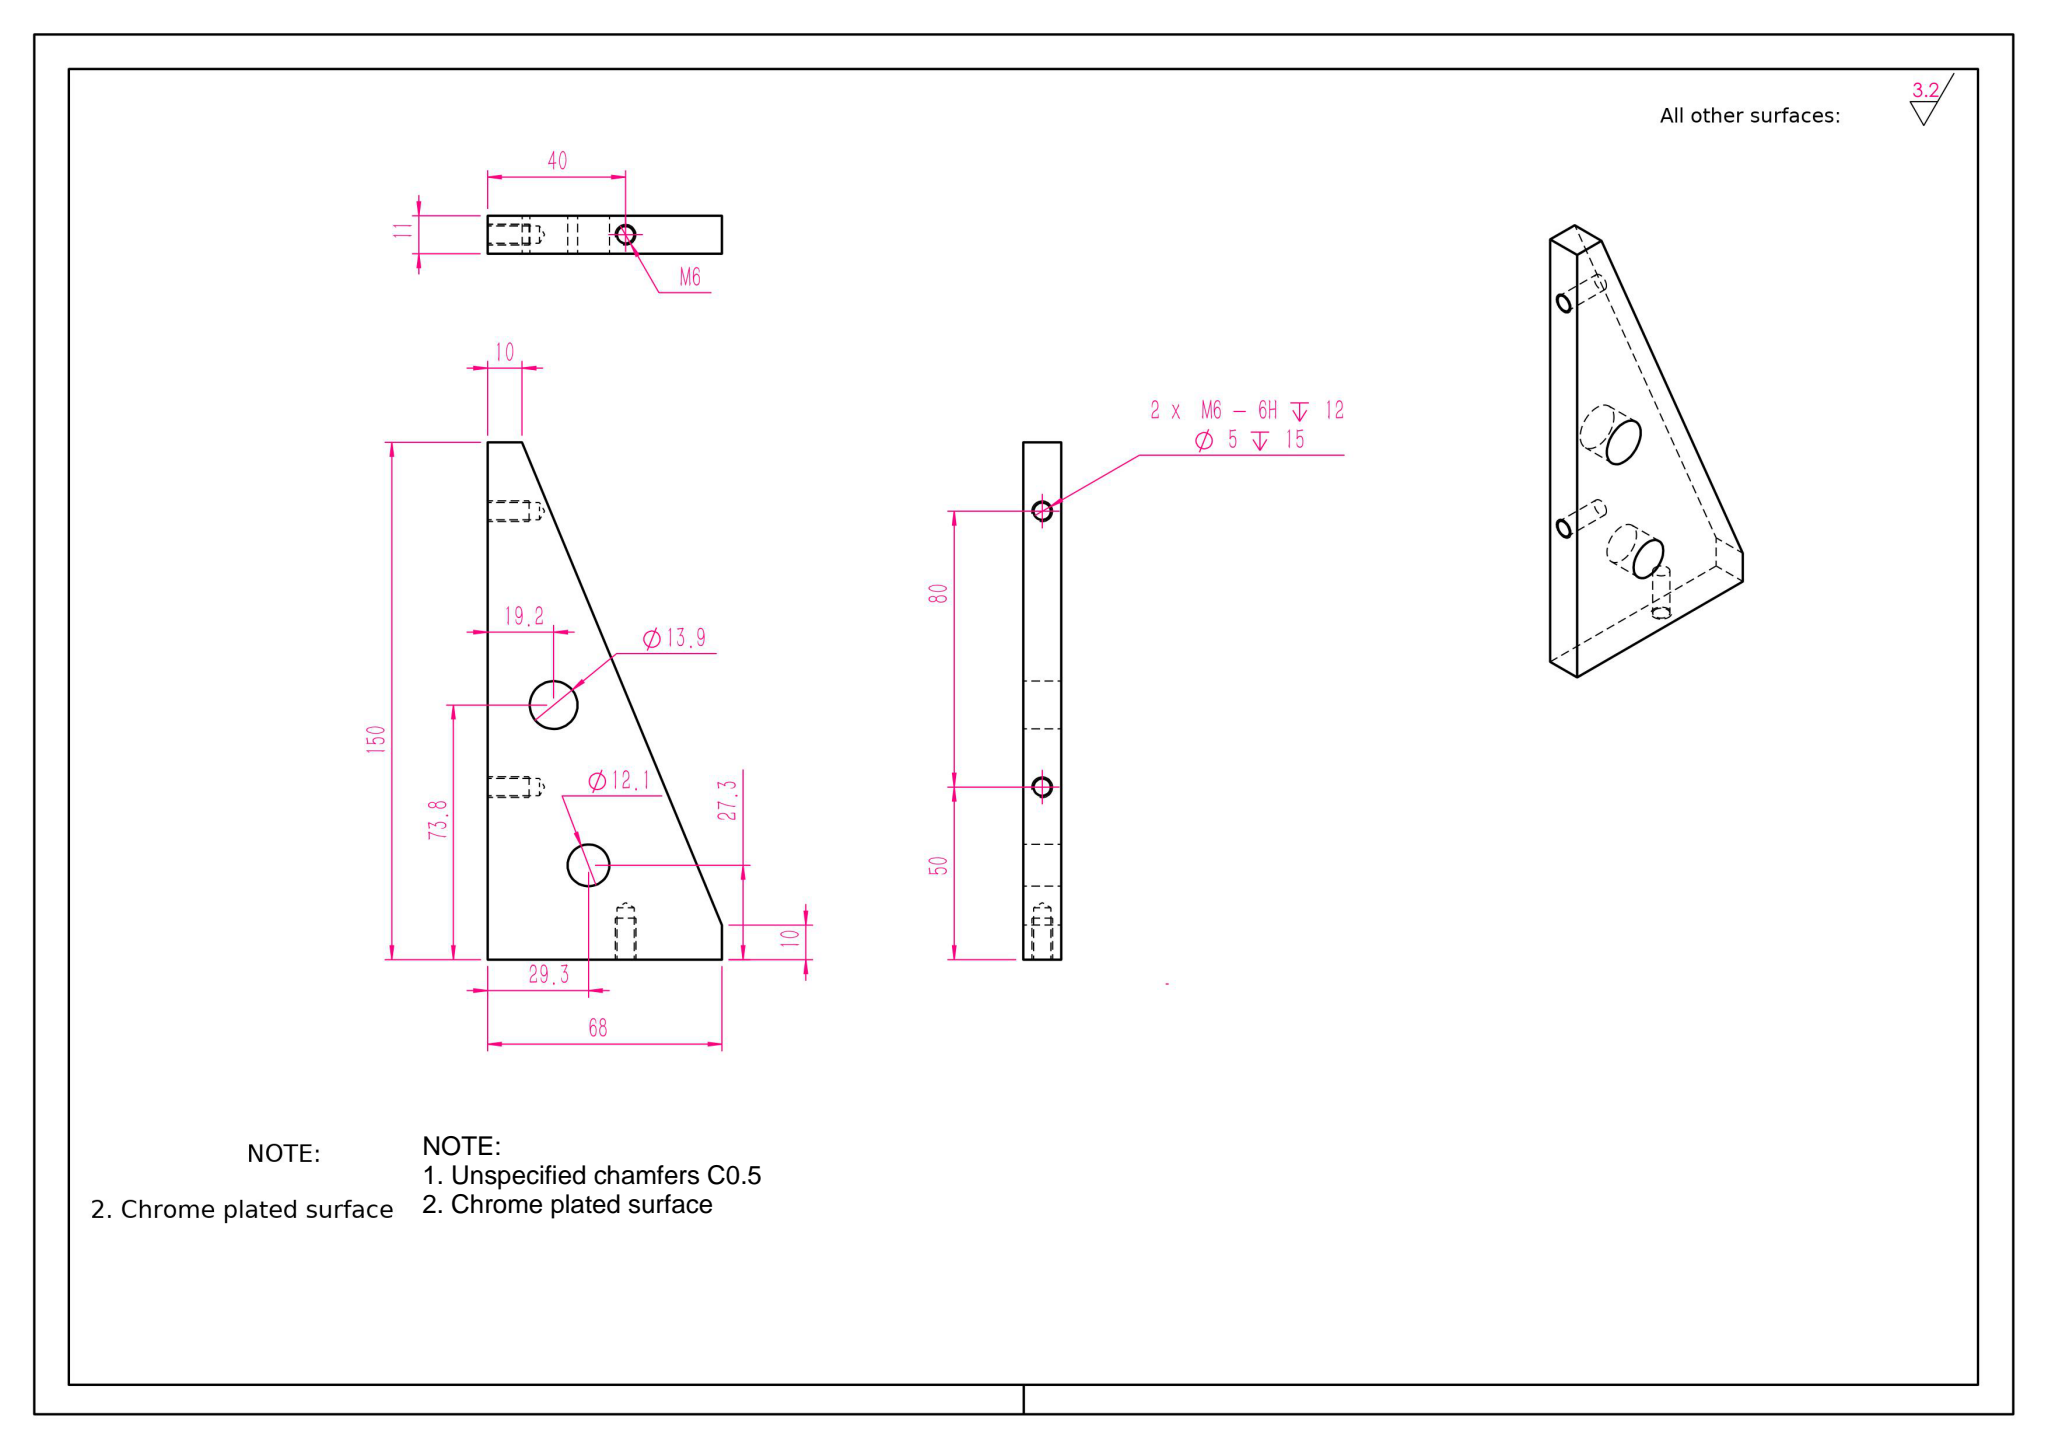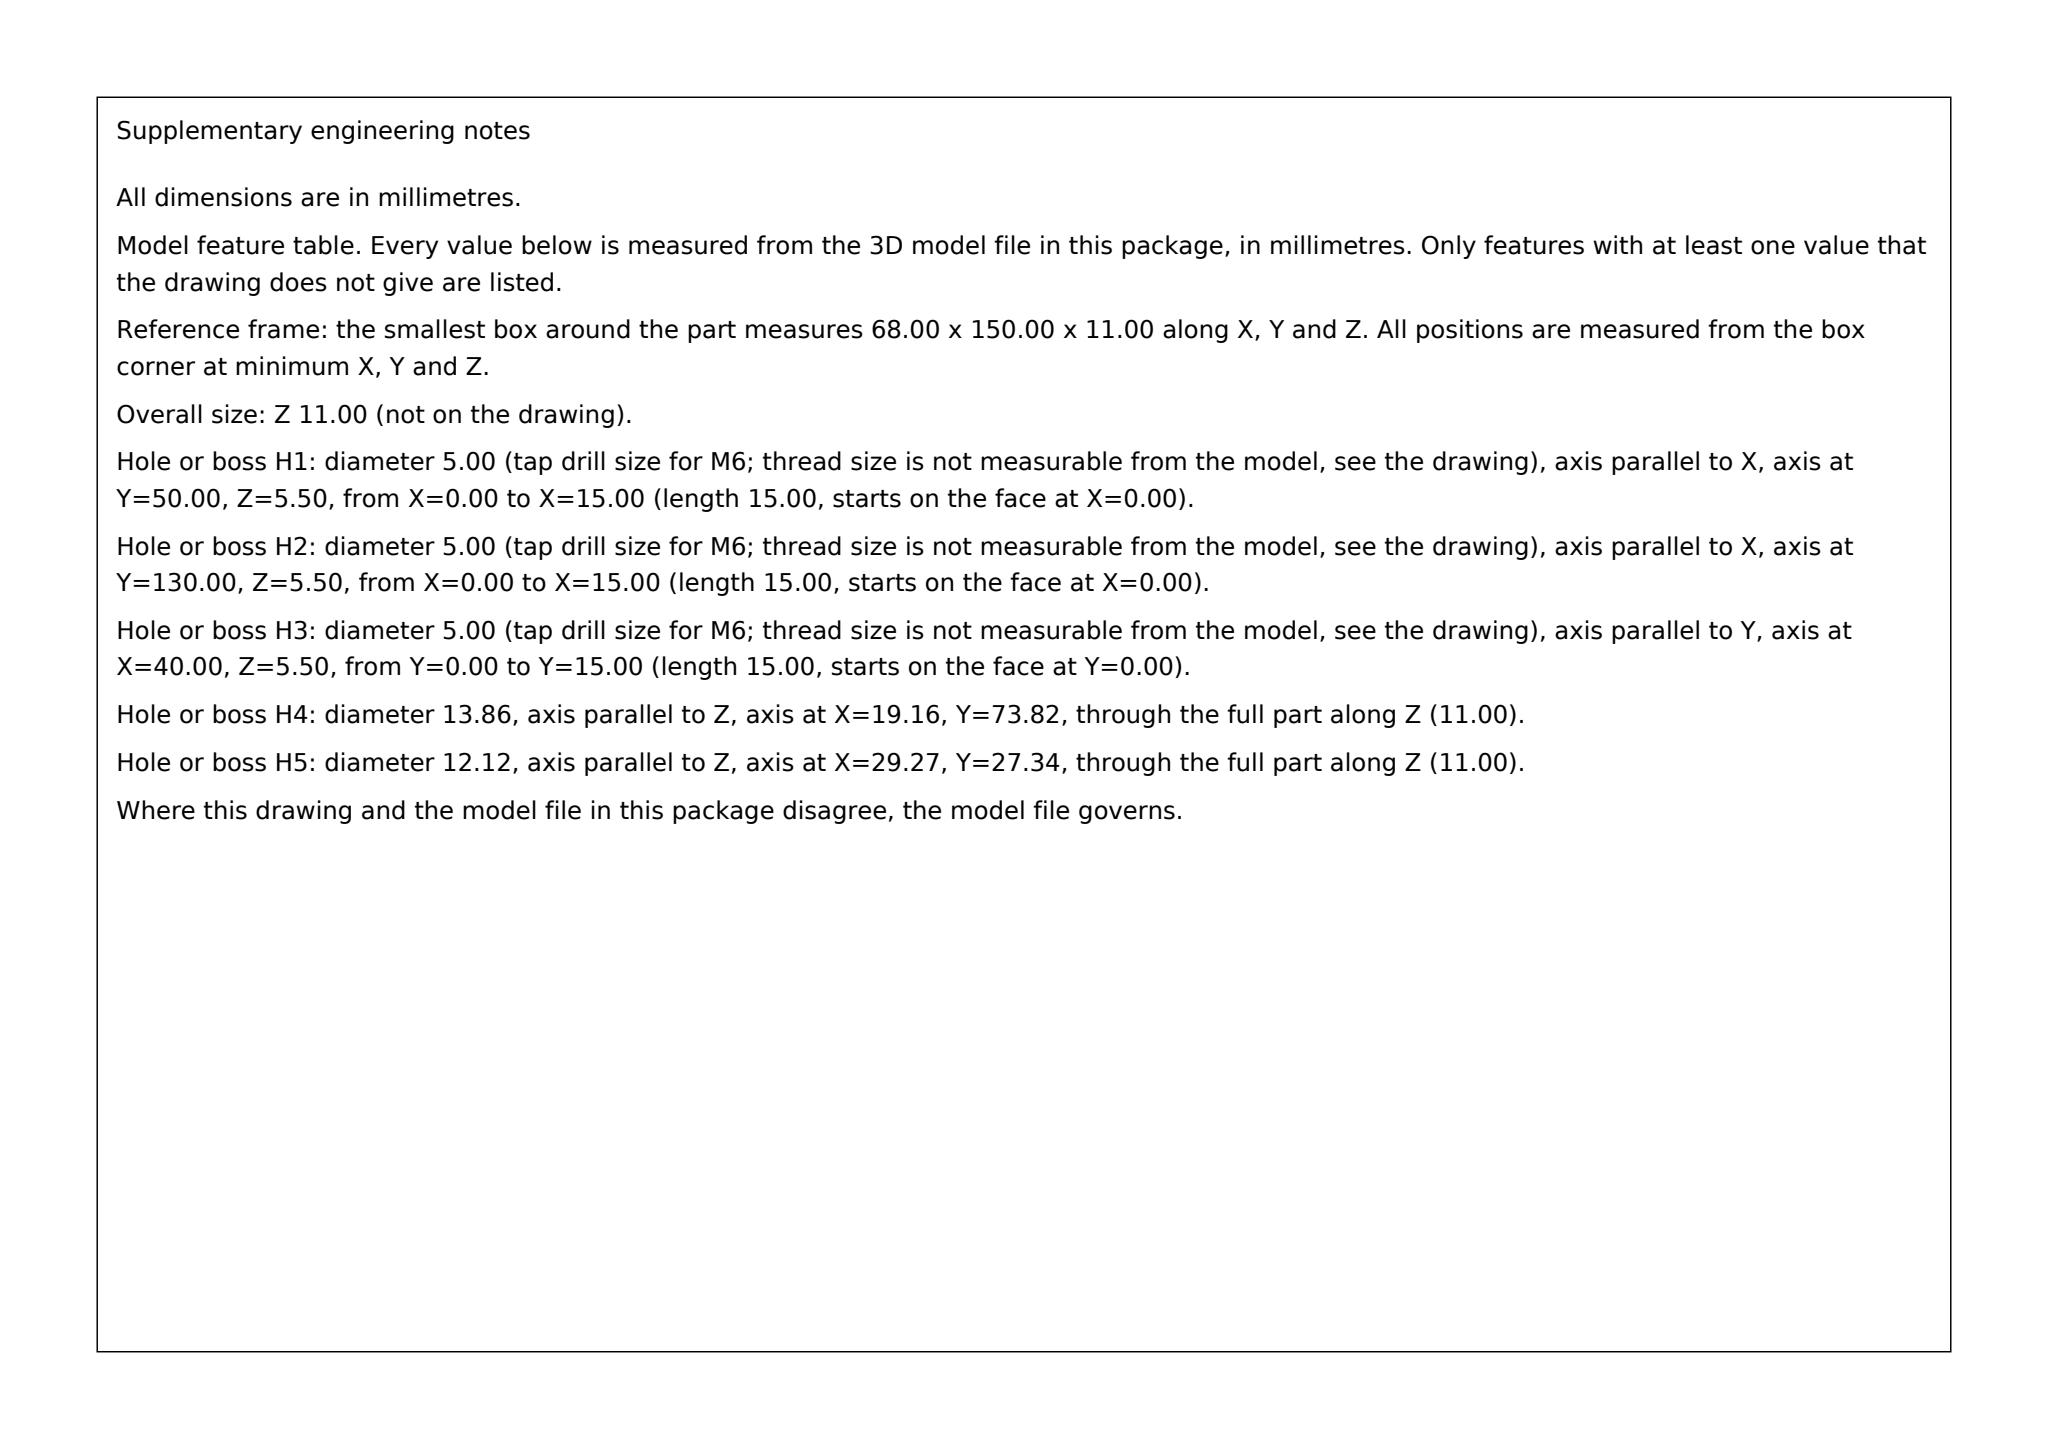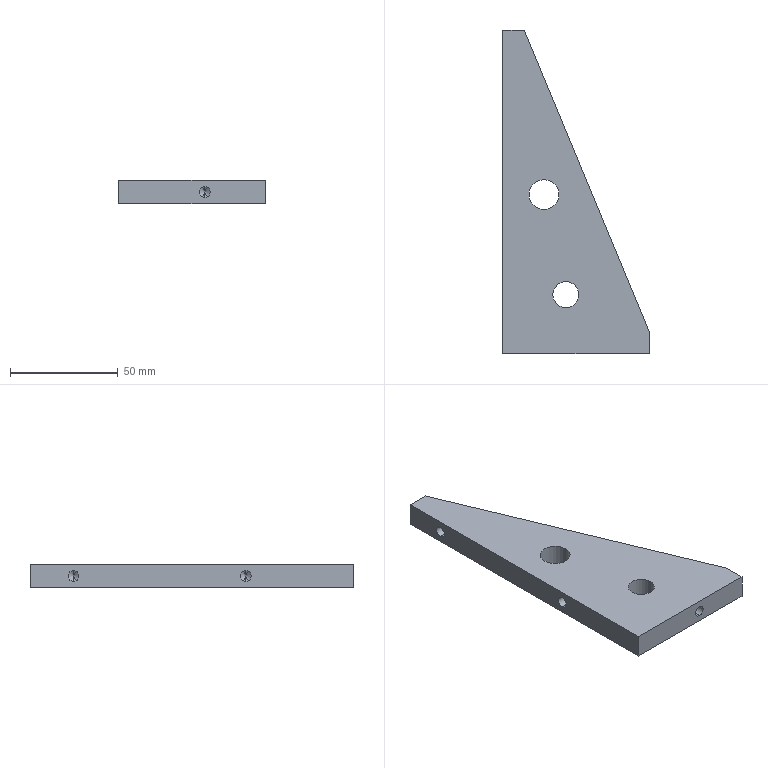Part | SolidWorks | mm | 1 solid | 23 faces | box 68 x 150 x 11 mm | volume 63698 mm3 | cylinder 10 | plane 7 | cone 6 | commonest cylinder face diameters 5 x6 12.125 x2 13.857 x2
build123d program:
from build123d import *

# Parameters (mm, degrees)
BOSS_EXTRUDE1_DEPTH   = 11
M6_TAPPED_HOLE1_D     = 5
M6_TAPPED_HOLE1_DEPTH = 15
M6_TAPPED_HOLE1_TIP   = 1.502
M6_TAPPED_HOLE2_D     = 5
M6_TAPPED_HOLE2_DEPTH = 15
M6_TAPPED_HOLE2_TIP   = 1.502
SKETCH8_R             = 6.063
SKETCH8_R_2           = 6.928
CUT_EXTRUDE1_DEPTH    = 80


with BuildPart() as part:
    # Sketch1 → Boss-Extrude1 (new body)
    with BuildSketch(Plane.XY):
        Polygon((0, 0), (68, 0), (68, 10), (10, 150), (0, 150), align=None)
    extrude(amount=BOSS_EXTRUDE1_DEPTH)

    # M6 Tapped Hole1
    with Locations(Plane(origin=(0, 0, 0), x_dir=(-1, 0, 0), z_dir=(0, -1, 0))):
        with Locations((-40, -5.5)):
            Hole(M6_TAPPED_HOLE1_D / 2, depth=M6_TAPPED_HOLE1_DEPTH)
            with Locations((0, 0, -(M6_TAPPED_HOLE1_DEPTH + M6_TAPPED_HOLE1_TIP / 2))):  # 118° drill point
                Cone(0, M6_TAPPED_HOLE1_D / 2, M6_TAPPED_HOLE1_TIP, mode=Mode.SUBTRACT)

    # M6 Tapped Hole2
    with Locations(Plane.ZY):
        with Locations((5.5, 130), (5.5, 50)):
            Hole(M6_TAPPED_HOLE2_D / 2, depth=M6_TAPPED_HOLE2_DEPTH)
            with Locations((0, 0, -(M6_TAPPED_HOLE2_DEPTH + M6_TAPPED_HOLE2_TIP / 2))):  # 118° drill point
                Cone(0, M6_TAPPED_HOLE2_D / 2, M6_TAPPED_HOLE2_TIP, mode=Mode.SUBTRACT)

    # Sketch8 → Cut-Extrude1 (cut)
    with BuildSketch(Plane.XY.offset(11)):
        with Locations((29.268, 27.343)):
            Circle(SKETCH8_R)
        with Locations((19.156, 73.817)):
            Circle(SKETCH8_R_2)
    extrude(amount=-CUT_EXTRUDE1_DEPTH, mode=Mode.SUBTRACT)


solid = part.part
STEP:
#1=CARTESIAN_POINT('',(23.206,27.343,0.));
#2=VERTEX_POINT('',#1);
#3=CARTESIAN_POINT('',(35.331,27.343,0.));
#4=VERTEX_POINT('',#3);
#5=CARTESIAN_POINT('',(29.268,27.343,0.));
#6=DIRECTION('',(0.,0.,1.));
#7=DIRECTION('',(1.,0.,0.));
#8=AXIS2_PLACEMENT_3D('',#5,#6,#7);
#9=CIRCLE('',#8,6.063);
#10=EDGE_CURVE('',#2,#4,#9,.T.);
#11=ORIENTED_EDGE('',*,*,#10,.F.);
#12=CARTESIAN_POINT('',(23.206,27.343,11.));
#13=VERTEX_POINT('',#12);
#14=CARTESIAN_POINT('',(23.206,27.343,-69.));
#15=DIRECTION('',(0.,0.,1.));
#16=VECTOR('',#15,1000.);
#17=LINE('',#14,#16);
#18=EDGE_CURVE('',#2,#13,#17,.T.);
#19=ORIENTED_EDGE('',*,*,#18,.T.);
#20=CARTESIAN_POINT('',(35.331,27.343,11.));
#21=VERTEX_POINT('',#20);
#22=CARTESIAN_POINT('',(29.268,27.343,11.));
#23=DIRECTION('',(0.,0.,1.));
#24=DIRECTION('',(1.,0.,0.));
#25=AXIS2_PLACEMENT_3D('',#22,#23,#24);
#26=CIRCLE('',#25,6.063);
#27=EDGE_CURVE('',#13,#21,#26,.T.);
#28=ORIENTED_EDGE('',*,*,#27,.T.);
#29=CARTESIAN_POINT('',(35.331,27.343,-69.));
#30=DIRECTION('',(0.,0.,1.));
#31=VECTOR('',#30,1000.);
#32=LINE('',#29,#31);
#33=EDGE_CURVE('',#4,#21,#32,.T.);
#34=ORIENTED_EDGE('',*,*,#33,.F.);
#35=EDGE_LOOP('',(#11,#19,#28,#34));
#36=FACE_OUTER_BOUND('',#35,.T.);
#37=CARTESIAN_POINT('',(29.268,27.343,-69.));
#38=DIRECTION('',(0.,0.,1.));
#39=DIRECTION('',(1.,0.,0.));
#40=AXIS2_PLACEMENT_3D('',#37,#38,#39);
#41=CYLINDRICAL_SURFACE('',#40,6.063);
#42=ADVANCED_FACE('',(#36),#41,.F.);
#43=CARTESIAN_POINT('',(12.228,73.817,0.));
#44=VERTEX_POINT('',#43);
#45=CARTESIAN_POINT('',(26.085,73.817,0.));
#46=VERTEX_POINT('',#45);
#47=CARTESIAN_POINT('',(19.156,73.817,0.));
#48=DIRECTION('',(0.,0.,1.));
#49=DIRECTION('',(1.,0.,0.));
#50=AXIS2_PLACEMENT_3D('',#47,#48,#49);
#51=CIRCLE('',#50,6.928);
#52=EDGE_CURVE('',#44,#46,#51,.T.);
#53=ORIENTED_EDGE('',*,*,#52,.F.);
#54=CARTESIAN_POINT('',(12.228,73.817,11.));
#55=VERTEX_POINT('',#54);
#56=CARTESIAN_POINT('',(12.228,73.817,-69.));
#57=DIRECTION('',(0.,0.,1.));
#58=VECTOR('',#57,1000.);
#59=LINE('',#56,#58);
#60=EDGE_CURVE('',#44,#55,#59,.T.);
#61=ORIENTED_EDGE('',*,*,#60,.T.);
#62=CARTESIAN_POINT('',(26.085,73.817,11.));
#63=VERTEX_POINT('',#62);
#64=CARTESIAN_POINT('',(19.156,73.817,11.));
#65=DIRECTION('',(0.,0.,1.));
#66=DIRECTION('',(1.,0.,0.));
#67=AXIS2_PLACEMENT_3D('',#64,#65,#66);
#68=CIRCLE('',#67,6.928);
#69=EDGE_CURVE('',#55,#63,#68,.T.);
#70=ORIENTED_EDGE('',*,*,#69,.T.);
#71=CARTESIAN_POINT('',(26.085,73.817,-69.));
#72=DIRECTION('',(0.,0.,1.));
#73=VECTOR('',#72,1000.);
#74=LINE('',#71,#73);
#75=EDGE_CURVE('',#46,#63,#74,.T.);
#76=ORIENTED_EDGE('',*,*,#75,.F.);
#77=EDGE_LOOP('',(#53,#61,#70,#76));
#78=FACE_OUTER_BOUND('',#77,.T.);
#79=CARTESIAN_POINT('',(19.156,73.817,-69.));
#80=DIRECTION('',(0.,0.,1.));
#81=DIRECTION('',(1.,0.,0.));
#82=AXIS2_PLACEMENT_3D('',#79,#80,#81);
#83=CYLINDRICAL_SURFACE('',#82,6.928);
#84=ADVANCED_FACE('',(#78),#83,.F.);
#85=CARTESIAN_POINT('',(15.,130.,3.));
#86=VERTEX_POINT('',#85);
#87=CARTESIAN_POINT('',(15.,130.,8.));
#88=VERTEX_POINT('',#87);
#89=CARTESIAN_POINT('',(15.,130.,5.5));
#90=DIRECTION('',(-1.,0.,0.));
#91=DIRECTION('',(0.,0.,1.));
#92=AXIS2_PLACEMENT_3D('',#89,#90,#91);
#93=CIRCLE('',#92,2.5);
#94=EDGE_CURVE('',#86,#88,#93,.T.);
#95=ORIENTED_EDGE('',*,*,#94,.F.);
#96=CARTESIAN_POINT('',(-0.,130.,3.));
#97=VERTEX_POINT('',#96);
#98=CARTESIAN_POINT('',(-0.,130.,3.));
#99=DIRECTION('',(-1.,0.,0.));
#100=VECTOR('',#99,1000.);
#101=LINE('',#98,#100);
#102=EDGE_CURVE('',#86,#97,#101,.T.);
#103=ORIENTED_EDGE('',*,*,#102,.T.);
#104=CARTESIAN_POINT('',(-0.,130.,8.));
#105=VERTEX_POINT('',#104);
#106=CARTESIAN_POINT('',(-0.,130.,5.5));
#107=DIRECTION('',(-1.,0.,0.));
#108=DIRECTION('',(0.,0.,1.));
#109=AXIS2_PLACEMENT_3D('',#106,#107,#108);
#110=CIRCLE('',#109,2.5);
#111=EDGE_CURVE('',#97,#105,#110,.T.);
#112=ORIENTED_EDGE('',*,*,#111,.T.);
#113=CARTESIAN_POINT('',(-0.,130.,8.));
#114=DIRECTION('',(-1.,0.,0.));
#115=VECTOR('',#114,1000.);
#116=LINE('',#113,#115);
#117=EDGE_CURVE('',#88,#105,#116,.T.);
#118=ORIENTED_EDGE('',*,*,#117,.F.);
#119=EDGE_LOOP('',(#95,#103,#112,#118));
#120=FACE_OUTER_BOUND('',#119,.T.);
#121=CARTESIAN_POINT('',(-0.,130.,5.5));
#122=DIRECTION('',(-1.,0.,0.));
#123=DIRECTION('',(0.,0.,1.));
#124=AXIS2_PLACEMENT_3D('',#121,#122,#123);
#125=CYLINDRICAL_SURFACE('',#124,2.5);
#126=ADVANCED_FACE('',(#120),#125,.F.);
#127=CARTESIAN_POINT('',(16.502,130.,5.5));
#128=VERTEX_POINT('',#127);
#129=CARTESIAN_POINT('',(15.,130.,8.));
#130=DIRECTION('',(-0.515,0.,0.8572));
#131=VECTOR('',#130,1000.);
#132=LINE('',#129,#131);
#133=EDGE_CURVE('',#128,#88,#132,.T.);
#134=ORIENTED_EDGE('',*,*,#133,.F.);
#135=CARTESIAN_POINT('',(15.,130.,3.));
#136=DIRECTION('',(-0.515,0.,-0.8572));
#137=VECTOR('',#136,1000.);
#138=LINE('',#135,#137);
#139=EDGE_CURVE('',#128,#86,#138,.T.);
#140=ORIENTED_EDGE('',*,*,#139,.T.);
#141=ORIENTED_EDGE('',*,*,#94,.T.);
#142=EDGE_LOOP('',(#134,#140,#141));
#143=FACE_OUTER_BOUND('',#142,.T.);
#144=CARTESIAN_POINT('',(15.,130.,5.5));
#145=DIRECTION('',(-1.,0.,0.));
#146=DIRECTION('',(0.,0.,1.));
#147=AXIS2_PLACEMENT_3D('',#144,#145,#146);
#148=CONICAL_SURFACE('',#147,2.5,1.03);
#149=ADVANCED_FACE('',(#143),#148,.F.);
#150=CARTESIAN_POINT('',(15.,50.,3.));
#151=VERTEX_POINT('',#150);
#152=CARTESIAN_POINT('',(15.,50.,8.));
#153=VERTEX_POINT('',#152);
#154=CARTESIAN_POINT('',(15.,50.,5.5));
#155=DIRECTION('',(-1.,0.,0.));
#156=DIRECTION('',(0.,0.,1.));
#157=AXIS2_PLACEMENT_3D('',#154,#155,#156);
#158=CIRCLE('',#157,2.5);
#159=EDGE_CURVE('',#151,#153,#158,.T.);
#160=ORIENTED_EDGE('',*,*,#159,.F.);
#161=CARTESIAN_POINT('',(-0.,50.,3.));
#162=VERTEX_POINT('',#161);
#163=CARTESIAN_POINT('',(-0.,50.,3.));
#164=DIRECTION('',(-1.,0.,0.));
#165=VECTOR('',#164,1000.);
#166=LINE('',#163,#165);
#167=EDGE_CURVE('',#151,#162,#166,.T.);
#168=ORIENTED_EDGE('',*,*,#167,.T.);
#169=CARTESIAN_POINT('',(-0.,50.,8.));
#170=VERTEX_POINT('',#169);
#171=CARTESIAN_POINT('',(-0.,50.,5.5));
#172=DIRECTION('',(-1.,0.,0.));
#173=DIRECTION('',(0.,0.,1.));
#174=AXIS2_PLACEMENT_3D('',#171,#172,#173);
#175=CIRCLE('',#174,2.5);
#176=EDGE_CURVE('',#162,#170,#175,.T.);
#177=ORIENTED_EDGE('',*,*,#176,.T.);
#178=CARTESIAN_POINT('',(-0.,50.,8.));
#179=DIRECTION('',(-1.,0.,0.));
#180=VECTOR('',#179,1000.);
#181=LINE('',#178,#180);
#182=EDGE_CURVE('',#153,#170,#181,.T.);
#183=ORIENTED_EDGE('',*,*,#182,.F.);
#184=EDGE_LOOP('',(#160,#168,#177,#183));
#185=FACE_OUTER_BOUND('',#184,.T.);
#186=CARTESIAN_POINT('',(-0.,50.,5.5));
#187=DIRECTION('',(-1.,0.,0.));
#188=DIRECTION('',(0.,0.,1.));
#189=AXIS2_PLACEMENT_3D('',#186,#187,#188);
#190=CYLINDRICAL_SURFACE('',#189,2.5);
#191=ADVANCED_FACE('',(#185),#190,.F.);
#192=CARTESIAN_POINT('',(16.502,50.,5.5));
#193=VERTEX_POINT('',#192);
#194=CARTESIAN_POINT('',(15.,50.,8.));
#195=DIRECTION('',(-0.515,0.,0.8572));
#196=VECTOR('',#195,1000.);
#197=LINE('',#194,#196);
#198=EDGE_CURVE('',#193,#153,#197,.T.);
#199=ORIENTED_EDGE('',*,*,#198,.F.);
#200=CARTESIAN_POINT('',(15.,50.,3.));
#201=DIRECTION('',(-0.515,0.,-0.8572));
#202=VECTOR('',#201,1000.);
#203=LINE('',#200,#202);
#204=EDGE_CURVE('',#193,#151,#203,.T.);
#205=ORIENTED_EDGE('',*,*,#204,.T.);
#206=ORIENTED_EDGE('',*,*,#159,.T.);
#207=EDGE_LOOP('',(#199,#205,#206));
#208=FACE_OUTER_BOUND('',#207,.T.);
#209=CARTESIAN_POINT('',(15.,50.,5.5));
#210=DIRECTION('',(-1.,0.,0.));
#211=DIRECTION('',(0.,0.,1.));
#212=AXIS2_PLACEMENT_3D('',#209,#210,#211);
#213=CONICAL_SURFACE('',#212,2.5,1.03);
#214=ADVANCED_FACE('',(#208),#213,.F.);
#215=CARTESIAN_POINT('',(40.,15.,8.));
#216=VERTEX_POINT('',#215);
#217=CARTESIAN_POINT('',(40.,15.,3.));
#218=VERTEX_POINT('',#217);
#219=CARTESIAN_POINT('',(40.,15.,5.5));
#220=DIRECTION('',(0.,-1.,0.));
#221=DIRECTION('',(0.,0.,-1.));
#222=AXIS2_PLACEMENT_3D('',#219,#220,#221);
#223=CIRCLE('',#222,2.5);
#224=EDGE_CURVE('',#216,#218,#223,.T.);
#225=ORIENTED_EDGE('',*,*,#224,.F.);
#226=CARTESIAN_POINT('',(40.,-0.,8.));
#227=VERTEX_POINT('',#226);
#228=CARTESIAN_POINT('',(40.,0.,8.));
#229=DIRECTION('',(0.,-1.,0.));
#230=VECTOR('',#229,1000.);
#231=LINE('',#228,#230);
#232=EDGE_CURVE('',#216,#227,#231,.T.);
#233=ORIENTED_EDGE('',*,*,#232,.T.);
#234=CARTESIAN_POINT('',(40.,-0.,3.));
#235=VERTEX_POINT('',#234);
#236=CARTESIAN_POINT('',(40.,-0.,5.5));
#237=DIRECTION('',(0.,-1.,0.));
#238=DIRECTION('',(0.,0.,-1.));
#239=AXIS2_PLACEMENT_3D('',#236,#237,#238);
#240=CIRCLE('',#239,2.5);
#241=EDGE_CURVE('',#227,#235,#240,.T.);
#242=ORIENTED_EDGE('',*,*,#241,.T.);
#243=CARTESIAN_POINT('',(40.,0.,3.));
#244=DIRECTION('',(0.,-1.,0.));
#245=VECTOR('',#244,1000.);
#246=LINE('',#243,#245);
#247=EDGE_CURVE('',#218,#235,#246,.T.);
#248=ORIENTED_EDGE('',*,*,#247,.F.);
#249=EDGE_LOOP('',(#225,#233,#242,#248));
#250=FACE_OUTER_BOUND('',#249,.T.);
#251=CARTESIAN_POINT('',(40.,0.,5.5));
#252=DIRECTION('',(0.,-1.,0.));
#253=DIRECTION('',(0.,0.,-1.));
#254=AXIS2_PLACEMENT_3D('',#251,#252,#253);
#255=CYLINDRICAL_SURFACE('',#254,2.5);
#256=ADVANCED_FACE('',(#250),#255,.F.);
#257=CARTESIAN_POINT('',(40.,16.502,5.5));
#258=VERTEX_POINT('',#257);
#259=CARTESIAN_POINT('',(40.,15.,3.));
#260=DIRECTION('',(0.,-0.515,-0.8572));
#261=VECTOR('',#260,1000.);
#262=LINE('',#259,#261);
#263=EDGE_CURVE('',#258,#218,#262,.T.);
#264=ORIENTED_EDGE('',*,*,#263,.F.);
#265=CARTESIAN_POINT('',(40.,15.,8.));
#266=DIRECTION('',(0.,-0.515,0.8572));
#267=VECTOR('',#266,1000.);
#268=LINE('',#265,#267);
#269=EDGE_CURVE('',#258,#216,#268,.T.);
#270=ORIENTED_EDGE('',*,*,#269,.T.);
#271=ORIENTED_EDGE('',*,*,#224,.T.);
#272=EDGE_LOOP('',(#264,#270,#271));
#273=FACE_OUTER_BOUND('',#272,.T.);
#274=CARTESIAN_POINT('',(40.,15.,5.5));
#275=DIRECTION('',(0.,-1.,0.));
#276=DIRECTION('',(0.,0.,-1.));
#277=AXIS2_PLACEMENT_3D('',#274,#275,#276);
#278=CONICAL_SURFACE('',#277,2.5,1.03);
#279=ADVANCED_FACE('',(#273),#278,.F.);
#280=CARTESIAN_POINT('',(-0.,130.,5.5));
#281=DIRECTION('',(-1.,0.,0.));
#282=DIRECTION('',(0.,0.,1.));
#283=AXIS2_PLACEMENT_3D('',#280,#281,#282);
#284=CIRCLE('',#283,2.5);
#285=EDGE_CURVE('',#105,#97,#284,.T.);
#286=ORIENTED_EDGE('',*,*,#285,.F.);
#287=ORIENTED_EDGE('',*,*,#111,.F.);
#288=EDGE_LOOP('',(#286,#287));
#289=FACE_BOUND('',#288,.T.);
#290=CARTESIAN_POINT('',(-0.,50.,5.5));
#291=DIRECTION('',(-1.,0.,0.));
#292=DIRECTION('',(0.,0.,1.));
#293=AXIS2_PLACEMENT_3D('',#290,#291,#292);
#294=CIRCLE('',#293,2.5);
#295=EDGE_CURVE('',#170,#162,#294,.T.);
#296=ORIENTED_EDGE('',*,*,#295,.F.);
#297=ORIENTED_EDGE('',*,*,#176,.F.);
#298=EDGE_LOOP('',(#296,#297));
#299=FACE_BOUND('',#298,.T.);
#300=CARTESIAN_POINT('',(-0.,150.,0.));
#301=VERTEX_POINT('',#300);
#302=CARTESIAN_POINT('',(0.,0.,0.));
#303=VERTEX_POINT('',#302);
#304=CARTESIAN_POINT('',(-0.,150.,0.));
#305=DIRECTION('',(0.,-1.,0.));
#306=VECTOR('',#305,1000.);
#307=LINE('',#304,#306);
#308=EDGE_CURVE('',#301,#303,#307,.T.);
#309=ORIENTED_EDGE('',*,*,#308,.T.);
#310=CARTESIAN_POINT('',(0.,0.,11.));
#311=VERTEX_POINT('',#310);
#312=CARTESIAN_POINT('',(0.,0.,11.));
#313=DIRECTION('',(0.,0.,-1.));
#314=VECTOR('',#313,1000.);
#315=LINE('',#312,#314);
#316=EDGE_CURVE('',#311,#303,#315,.T.);
#317=ORIENTED_EDGE('',*,*,#316,.F.);
#318=CARTESIAN_POINT('',(-0.,150.,11.));
#319=VERTEX_POINT('',#318);
#320=CARTESIAN_POINT('',(-0.,150.,11.));
#321=DIRECTION('',(0.,-1.,0.));
#322=VECTOR('',#321,1000.);
#323=LINE('',#320,#322);
#324=EDGE_CURVE('',#319,#311,#323,.T.);
#325=ORIENTED_EDGE('',*,*,#324,.F.);
#326=CARTESIAN_POINT('',(-0.,150.,11.));
#327=DIRECTION('',(0.,0.,-1.));
#328=VECTOR('',#327,1000.);
#329=LINE('',#326,#328);
#330=EDGE_CURVE('',#319,#301,#329,.T.);
#331=ORIENTED_EDGE('',*,*,#330,.T.);
#332=EDGE_LOOP('',(#309,#317,#325,#331));
#333=FACE_OUTER_BOUND('',#332,.T.);
#334=CARTESIAN_POINT('',(-0.,150.,11.));
#335=DIRECTION('',(1.,0.,0.));
#336=DIRECTION('',(-0.,1.,0.));
#337=AXIS2_PLACEMENT_3D('',#334,#335,#336);
#338=PLANE('',#337);
#339=ADVANCED_FACE('',(#289,#299,#333),#338,.F.);
#340=CARTESIAN_POINT('',(40.,-0.,5.5));
#341=DIRECTION('',(0.,-1.,0.));
#342=DIRECTION('',(0.,0.,-1.));
#343=AXIS2_PLACEMENT_3D('',#340,#341,#342);
#344=CIRCLE('',#343,2.5);
#345=EDGE_CURVE('',#235,#227,#344,.T.);
#346=ORIENTED_EDGE('',*,*,#345,.F.);
#347=ORIENTED_EDGE('',*,*,#241,.F.);
#348=EDGE_LOOP('',(#346,#347));
#349=FACE_BOUND('',#348,.T.);
#350=CARTESIAN_POINT('',(68.,0.,0.));
#351=VERTEX_POINT('',#350);
#352=CARTESIAN_POINT('',(0.,0.,0.));
#353=DIRECTION('',(1.,0.,0.));
#354=VECTOR('',#353,1000.);
#355=LINE('',#352,#354);
#356=EDGE_CURVE('',#303,#351,#355,.T.);
#357=ORIENTED_EDGE('',*,*,#356,.T.);
#358=CARTESIAN_POINT('',(68.,0.,11.));
#359=VERTEX_POINT('',#358);
#360=CARTESIAN_POINT('',(68.,0.,11.));
#361=DIRECTION('',(0.,0.,-1.));
#362=VECTOR('',#361,1000.);
#363=LINE('',#360,#362);
#364=EDGE_CURVE('',#359,#351,#363,.T.);
#365=ORIENTED_EDGE('',*,*,#364,.F.);
#366=CARTESIAN_POINT('',(0.,0.,11.));
#367=DIRECTION('',(1.,0.,0.));
#368=VECTOR('',#367,1000.);
#369=LINE('',#366,#368);
#370=EDGE_CURVE('',#311,#359,#369,.T.);
#371=ORIENTED_EDGE('',*,*,#370,.F.);
#372=ORIENTED_EDGE('',*,*,#316,.T.);
#373=EDGE_LOOP('',(#357,#365,#371,#372));
#374=FACE_OUTER_BOUND('',#373,.T.);
#375=CARTESIAN_POINT('',(0.,0.,11.));
#376=DIRECTION('',(0.,1.,0.));
#377=DIRECTION('',(0.,0.,1.));
#378=AXIS2_PLACEMENT_3D('',#375,#376,#377);
#379=PLANE('',#378);
#380=ADVANCED_FACE('',(#349,#374),#379,.F.);
#381=CARTESIAN_POINT('',(68.,10.,0.));
#382=VERTEX_POINT('',#381);
#383=CARTESIAN_POINT('',(68.,0.,0.));
#384=DIRECTION('',(0.,1.,0.));
#385=VECTOR('',#384,1000.);
#386=LINE('',#383,#385);
#387=EDGE_CURVE('',#351,#382,#386,.T.);
#388=ORIENTED_EDGE('',*,*,#387,.T.);
#389=CARTESIAN_POINT('',(68.,10.,11.));
#390=VERTEX_POINT('',#389);
#391=CARTESIAN_POINT('',(68.,10.,11.));
#392=DIRECTION('',(0.,0.,-1.));
#393=VECTOR('',#392,1000.);
#394=LINE('',#391,#393);
#395=EDGE_CURVE('',#390,#382,#394,.T.);
#396=ORIENTED_EDGE('',*,*,#395,.F.);
#397=CARTESIAN_POINT('',(68.,0.,11.));
#398=DIRECTION('',(0.,1.,0.));
#399=VECTOR('',#398,1000.);
#400=LINE('',#397,#399);
#401=EDGE_CURVE('',#359,#390,#400,.T.);
#402=ORIENTED_EDGE('',*,*,#401,.F.);
#403=ORIENTED_EDGE('',*,*,#364,.T.);
#404=EDGE_LOOP('',(#388,#396,#402,#403));
#405=FACE_OUTER_BOUND('',#404,.T.);
#406=CARTESIAN_POINT('',(68.,0.,11.));
#407=DIRECTION('',(-1.,0.,0.));
#408=DIRECTION('',(0.,0.,1.));
#409=AXIS2_PLACEMENT_3D('',#406,#407,#408);
#410=PLANE('',#409);
#411=ADVANCED_FACE('',(#405),#410,.F.);
#412=CARTESIAN_POINT('',(10.,150.,0.));
#413=VERTEX_POINT('',#412);
#414=CARTESIAN_POINT('',(68.,10.,0.));
#415=DIRECTION('',(-0.3827,0.9239,0.));
#416=VECTOR('',#415,1000.);
#417=LINE('',#414,#416);
#418=EDGE_CURVE('',#382,#413,#417,.T.);
#419=ORIENTED_EDGE('',*,*,#418,.T.);
#420=CARTESIAN_POINT('',(10.,150.,11.));
#421=VERTEX_POINT('',#420);
#422=CARTESIAN_POINT('',(10.,150.,11.));
#423=DIRECTION('',(0.,0.,-1.));
#424=VECTOR('',#423,1000.);
#425=LINE('',#422,#424);
#426=EDGE_CURVE('',#421,#413,#425,.T.);
#427=ORIENTED_EDGE('',*,*,#426,.F.);
#428=CARTESIAN_POINT('',(68.,10.,11.));
#429=DIRECTION('',(-0.3827,0.9239,0.));
#430=VECTOR('',#429,1000.);
#431=LINE('',#428,#430);
#432=EDGE_CURVE('',#390,#421,#431,.T.);
#433=ORIENTED_EDGE('',*,*,#432,.F.);
#434=ORIENTED_EDGE('',*,*,#395,.T.);
#435=EDGE_LOOP('',(#419,#427,#433,#434));
#436=FACE_OUTER_BOUND('',#435,.T.);
#437=CARTESIAN_POINT('',(68.,10.,11.));
#438=DIRECTION('',(-0.9239,-0.3827,0.));
#439=DIRECTION('',(0.3827,-0.9239,0.));
#440=AXIS2_PLACEMENT_3D('',#437,#438,#439);
#441=PLANE('',#440);
#442=ADVANCED_FACE('',(#436),#441,.F.);
#443=CARTESIAN_POINT('',(10.,150.,0.));
#444=DIRECTION('',(-1.,0.,0.));
#445=VECTOR('',#444,1000.);
#446=LINE('',#443,#445);
#447=EDGE_CURVE('',#413,#301,#446,.T.);
#448=ORIENTED_EDGE('',*,*,#447,.T.);
#449=ORIENTED_EDGE('',*,*,#330,.F.);
#450=CARTESIAN_POINT('',(10.,150.,11.));
#451=DIRECTION('',(-1.,0.,0.));
#452=VECTOR('',#451,1000.);
#453=LINE('',#450,#452);
#454=EDGE_CURVE('',#421,#319,#453,.T.);
#455=ORIENTED_EDGE('',*,*,#454,.F.);
#456=ORIENTED_EDGE('',*,*,#426,.T.);
#457=EDGE_LOOP('',(#448,#449,#455,#456));
#458=FACE_OUTER_BOUND('',#457,.T.);
#459=CARTESIAN_POINT('',(10.,150.,11.));
#460=DIRECTION('',(0.,-1.,0.));
#461=DIRECTION('',(0.,0.,-1.));
#462=AXIS2_PLACEMENT_3D('',#459,#460,#461);
#463=PLANE('',#462);
#464=ADVANCED_FACE('',(#458),#463,.F.);
#465=CARTESIAN_POINT('',(29.268,27.343,11.));
#466=DIRECTION('',(0.,0.,1.));
#467=DIRECTION('',(1.,0.,0.));
#468=AXIS2_PLACEMENT_3D('',#465,#466,#467);
#469=CIRCLE('',#468,6.063);
#470=EDGE_CURVE('',#21,#13,#469,.T.);
#471=ORIENTED_EDGE('',*,*,#470,.F.);
#472=ORIENTED_EDGE('',*,*,#27,.F.);
#473=EDGE_LOOP('',(#471,#472));
#474=FACE_BOUND('',#473,.T.);
#475=CARTESIAN_POINT('',(19.156,73.817,11.));
#476=DIRECTION('',(0.,0.,1.));
#477=DIRECTION('',(1.,0.,0.));
#478=AXIS2_PLACEMENT_3D('',#475,#476,#477);
#479=CIRCLE('',#478,6.928);
#480=EDGE_CURVE('',#63,#55,#479,.T.);
#481=ORIENTED_EDGE('',*,*,#480,.F.);
#482=ORIENTED_EDGE('',*,*,#69,.F.);
#483=EDGE_LOOP('',(#481,#482));
#484=FACE_BOUND('',#483,.T.);
#485=ORIENTED_EDGE('',*,*,#324,.T.);
#486=ORIENTED_EDGE('',*,*,#370,.T.);
#487=ORIENTED_EDGE('',*,*,#401,.T.);
#488=ORIENTED_EDGE('',*,*,#432,.T.);
#489=ORIENTED_EDGE('',*,*,#454,.T.);
#490=EDGE_LOOP('',(#485,#486,#487,#488,#489));
#491=FACE_OUTER_BOUND('',#490,.T.);
#492=CARTESIAN_POINT('',(0.,0.,11.));
#493=DIRECTION('',(0.,0.,1.));
#494=DIRECTION('',(1.,0.,0.));
#495=AXIS2_PLACEMENT_3D('',#492,#493,#494);
#496=PLANE('',#495);
#497=ADVANCED_FACE('',(#474,#484,#491),#496,.T.);
#498=CARTESIAN_POINT('',(29.268,27.343,0.));
#499=DIRECTION('',(0.,0.,1.));
#500=DIRECTION('',(1.,0.,0.));
#501=AXIS2_PLACEMENT_3D('',#498,#499,#500);
#502=CIRCLE('',#501,6.063);
#503=EDGE_CURVE('',#4,#2,#502,.T.);
#504=ORIENTED_EDGE('',*,*,#503,.T.);
#505=ORIENTED_EDGE('',*,*,#10,.T.);
#506=EDGE_LOOP('',(#504,#505));
#507=FACE_BOUND('',#506,.T.);
#508=CARTESIAN_POINT('',(19.156,73.817,0.));
#509=DIRECTION('',(0.,0.,1.));
#510=DIRECTION('',(1.,0.,0.));
#511=AXIS2_PLACEMENT_3D('',#508,#509,#510);
#512=CIRCLE('',#511,6.928);
#513=EDGE_CURVE('',#46,#44,#512,.T.);
#514=ORIENTED_EDGE('',*,*,#513,.T.);
#515=ORIENTED_EDGE('',*,*,#52,.T.);
#516=EDGE_LOOP('',(#514,#515));
#517=FACE_BOUND('',#516,.T.);
#518=ORIENTED_EDGE('',*,*,#308,.F.);
#519=ORIENTED_EDGE('',*,*,#447,.F.);
#520=ORIENTED_EDGE('',*,*,#418,.F.);
#521=ORIENTED_EDGE('',*,*,#387,.F.);
#522=ORIENTED_EDGE('',*,*,#356,.F.);
#523=EDGE_LOOP('',(#518,#519,#520,#521,#522));
#524=FACE_OUTER_BOUND('',#523,.T.);
#525=CARTESIAN_POINT('',(0.,0.,0.));
#526=DIRECTION('',(0.,0.,1.));
#527=DIRECTION('',(1.,0.,0.));
#528=AXIS2_PLACEMENT_3D('',#525,#526,#527);
#529=PLANE('',#528);
#530=ADVANCED_FACE('',(#507,#517,#524),#529,.F.);
#531=ORIENTED_EDGE('',*,*,#269,.F.);
#532=ORIENTED_EDGE('',*,*,#263,.T.);
#533=CARTESIAN_POINT('',(40.,15.,5.5));
#534=DIRECTION('',(0.,-1.,0.));
#535=DIRECTION('',(0.,0.,-1.));
#536=AXIS2_PLACEMENT_3D('',#533,#534,#535);
#537=CIRCLE('',#536,2.5);
#538=EDGE_CURVE('',#218,#216,#537,.T.);
#539=ORIENTED_EDGE('',*,*,#538,.T.);
#540=EDGE_LOOP('',(#531,#532,#539));
#541=FACE_OUTER_BOUND('',#540,.T.);
#542=CARTESIAN_POINT('',(40.,15.,5.5));
#543=DIRECTION('',(0.,-1.,0.));
#544=DIRECTION('',(0.,0.,-1.));
#545=AXIS2_PLACEMENT_3D('',#542,#543,#544);
#546=CONICAL_SURFACE('',#545,2.5,1.03);
#547=ADVANCED_FACE('',(#541),#546,.F.);
#548=ORIENTED_EDGE('',*,*,#232,.F.);
#549=ORIENTED_EDGE('',*,*,#538,.F.);
#550=ORIENTED_EDGE('',*,*,#247,.T.);
#551=ORIENTED_EDGE('',*,*,#345,.T.);
#552=EDGE_LOOP('',(#548,#549,#550,#551));
#553=FACE_OUTER_BOUND('',#552,.T.);
#554=CARTESIAN_POINT('',(40.,0.,5.5));
#555=DIRECTION('',(0.,-1.,0.));
#556=DIRECTION('',(0.,0.,-1.));
#557=AXIS2_PLACEMENT_3D('',#554,#555,#556);
#558=CYLINDRICAL_SURFACE('',#557,2.5);
#559=ADVANCED_FACE('',(#553),#558,.F.);
#560=ORIENTED_EDGE('',*,*,#204,.F.);
#561=ORIENTED_EDGE('',*,*,#198,.T.);
#562=CARTESIAN_POINT('',(15.,50.,5.5));
#563=DIRECTION('',(-1.,0.,0.));
#564=DIRECTION('',(0.,0.,1.));
#565=AXIS2_PLACEMENT_3D('',#562,#563,#564);
#566=CIRCLE('',#565,2.5);
#567=EDGE_CURVE('',#153,#151,#566,.T.);
#568=ORIENTED_EDGE('',*,*,#567,.T.);
#569=EDGE_LOOP('',(#560,#561,#568));
#570=FACE_OUTER_BOUND('',#569,.T.);
#571=CARTESIAN_POINT('',(15.,50.,5.5));
#572=DIRECTION('',(-1.,0.,0.));
#573=DIRECTION('',(0.,0.,1.));
#574=AXIS2_PLACEMENT_3D('',#571,#572,#573);
#575=CONICAL_SURFACE('',#574,2.5,1.03);
#576=ADVANCED_FACE('',(#570),#575,.F.);
#577=ORIENTED_EDGE('',*,*,#167,.F.);
#578=ORIENTED_EDGE('',*,*,#567,.F.);
#579=ORIENTED_EDGE('',*,*,#182,.T.);
#580=ORIENTED_EDGE('',*,*,#295,.T.);
#581=EDGE_LOOP('',(#577,#578,#579,#580));
#582=FACE_OUTER_BOUND('',#581,.T.);
#583=CARTESIAN_POINT('',(-0.,50.,5.5));
#584=DIRECTION('',(-1.,0.,0.));
#585=DIRECTION('',(0.,0.,1.));
#586=AXIS2_PLACEMENT_3D('',#583,#584,#585);
#587=CYLINDRICAL_SURFACE('',#586,2.5);
#588=ADVANCED_FACE('',(#582),#587,.F.);
#589=ORIENTED_EDGE('',*,*,#139,.F.);
#590=ORIENTED_EDGE('',*,*,#133,.T.);
#591=CARTESIAN_POINT('',(15.,130.,5.5));
#592=DIRECTION('',(-1.,0.,0.));
#593=DIRECTION('',(0.,0.,1.));
#594=AXIS2_PLACEMENT_3D('',#591,#592,#593);
#595=CIRCLE('',#594,2.5);
#596=EDGE_CURVE('',#88,#86,#595,.T.);
#597=ORIENTED_EDGE('',*,*,#596,.T.);
#598=EDGE_LOOP('',(#589,#590,#597));
#599=FACE_OUTER_BOUND('',#598,.T.);
#600=CARTESIAN_POINT('',(15.,130.,5.5));
#601=DIRECTION('',(-1.,0.,0.));
#602=DIRECTION('',(0.,0.,1.));
#603=AXIS2_PLACEMENT_3D('',#600,#601,#602);
#604=CONICAL_SURFACE('',#603,2.5,1.03);
#605=ADVANCED_FACE('',(#599),#604,.F.);
#606=ORIENTED_EDGE('',*,*,#102,.F.);
#607=ORIENTED_EDGE('',*,*,#596,.F.);
#608=ORIENTED_EDGE('',*,*,#117,.T.);
#609=ORIENTED_EDGE('',*,*,#285,.T.);
#610=EDGE_LOOP('',(#606,#607,#608,#609));
#611=FACE_OUTER_BOUND('',#610,.T.);
#612=CARTESIAN_POINT('',(-0.,130.,5.5));
#613=DIRECTION('',(-1.,0.,0.));
#614=DIRECTION('',(0.,0.,1.));
#615=AXIS2_PLACEMENT_3D('',#612,#613,#614);
#616=CYLINDRICAL_SURFACE('',#615,2.5);
#617=ADVANCED_FACE('',(#611),#616,.F.);
#618=ORIENTED_EDGE('',*,*,#60,.F.);
#619=ORIENTED_EDGE('',*,*,#513,.F.);
#620=ORIENTED_EDGE('',*,*,#75,.T.);
#621=ORIENTED_EDGE('',*,*,#480,.T.);
#622=EDGE_LOOP('',(#618,#619,#620,#621));
#623=FACE_OUTER_BOUND('',#622,.T.);
#624=CARTESIAN_POINT('',(19.156,73.817,-69.));
#625=DIRECTION('',(0.,0.,1.));
#626=DIRECTION('',(1.,0.,0.));
#627=AXIS2_PLACEMENT_3D('',#624,#625,#626);
#628=CYLINDRICAL_SURFACE('',#627,6.928);
#629=ADVANCED_FACE('',(#623),#628,.F.);
#630=ORIENTED_EDGE('',*,*,#18,.F.);
#631=ORIENTED_EDGE('',*,*,#503,.F.);
#632=ORIENTED_EDGE('',*,*,#33,.T.);
#633=ORIENTED_EDGE('',*,*,#470,.T.);
#634=EDGE_LOOP('',(#630,#631,#632,#633));
#635=FACE_OUTER_BOUND('',#634,.T.);
#636=CARTESIAN_POINT('',(29.268,27.343,-69.));
#637=DIRECTION('',(0.,0.,1.));
#638=DIRECTION('',(1.,0.,0.));
#639=AXIS2_PLACEMENT_3D('',#636,#637,#638);
#640=CYLINDRICAL_SURFACE('',#639,6.063);
#641=ADVANCED_FACE('',(#635),#640,.F.);
#642=CLOSED_SHELL('',(#42,#84,#126,#149,#191,#214,#256,#279,#339,#380,#411,#442,#464,#497,#530,#547,#559,#576,#588,#605,#617,#629,#641));
#643=MANIFOLD_SOLID_BREP('',#642);
#644=CARTESIAN_POINT('',(0.,0.,0.));
#645=DIRECTION('',(0.,0.,1.));
#646=DIRECTION('',(1.,0.,0.));
#647=AXIS2_PLACEMENT_3D('',#644,#645,#646);
#648=(LENGTH_UNIT()NAMED_UNIT(*)SI_UNIT(.MILLI.,.METRE.));
#649=UNCERTAINTY_MEASURE_WITH_UNIT(LENGTH_MEASURE(0.00001),#648,'','');
#650=(NAMED_UNIT(*)PLANE_ANGLE_UNIT()SI_UNIT($,.RADIAN.));
#651=(NAMED_UNIT(*)SI_UNIT($,.STERADIAN.)SOLID_ANGLE_UNIT());
#652=(GEOMETRIC_REPRESENTATION_CONTEXT(3)GLOBAL_UNCERTAINTY_ASSIGNED_CONTEXT((#649))GLOBAL_UNIT_ASSIGNED_CONTEXT((#648,#650,#651))REPRESENTATION_CONTEXT('',''));
#653=ADVANCED_BREP_SHAPE_REPRESENTATION('',(#643,#647),#652);